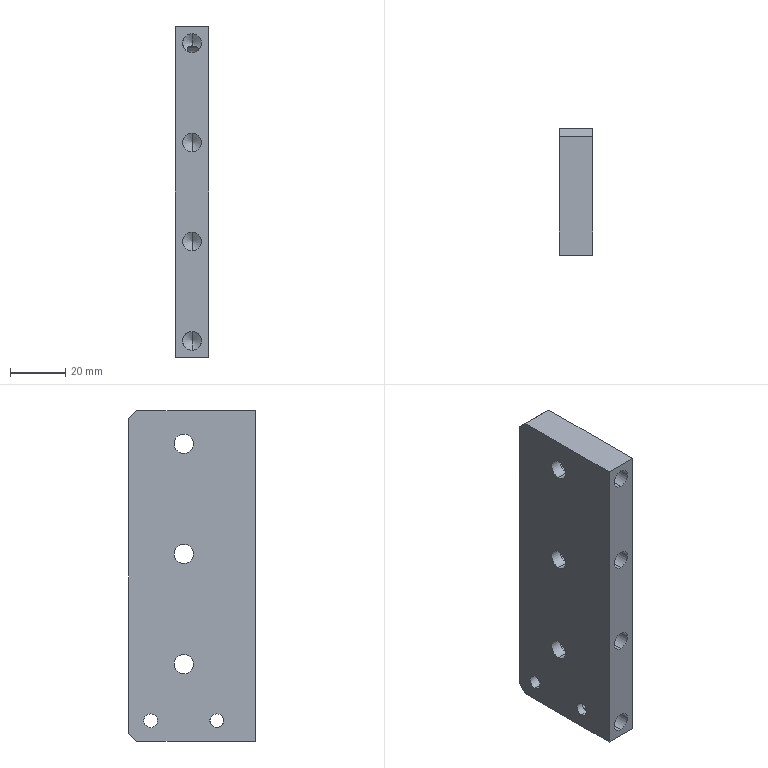Component | SolidWorks | ConveyorSideFixedLargePlateOne-2 | 1 solid | 43 faces | box 12 x 46 x 120 mm | volume 59730 mm3 | cylinder 24 | plane 11 | cone 8 | commonest cylinder face diameters 6.8 x8 11 x6 7 x6 5 x4 | material Plain Carbon Steel
build123d program:
from build123d import *

# Parameters (mm, degrees)
SKETCH1_W                                            = 120
SKETCH1_H                                            = 46
BOSS_EXTRUDE1_DEPTH                                  = 12
M8_TAPPED_HOLE1_D                                    = 6.8
M8_TAPPED_HOLE1_DEPTH                                = 22.25
M8_TAPPED_HOLE1_TIP                                  = 2.043
SKETCH4_R                                            = 3.5
CUT_EXTRUDE1_DEPTH                                   = 66.368
M6_TAPPED_HOLE1_D                                    = 5
HOLE_SIZE_ACCORDING_TO_TYPE_1_OF_HEXAGON_D           = 6.6
HOLE_SIZE_ACCORDING_TO_TYPE_1_OF_HEXAGON_CBORE_D     = 11
HOLE_SIZE_ACCORDING_TO_TYPE_1_OF_HEXAGON_CBORE_DEPTH = 7.8
CHAMFER1_SIZE                                        = 3


with BuildPart() as part:
    # Sketch1 → Boss-Extrude1 (new body)
    with BuildSketch(Plane(origin=(0, 0, 0), x_dir=(0, 0, -1), z_dir=(1, 0, 0))):
        Rectangle(SKETCH1_W, SKETCH1_H)
    extrude(amount=BOSS_EXTRUDE1_DEPTH)

    # M8 Tapped Hole1
    with Locations(Plane(origin=(0, -23, 0), x_dir=(-1, 0, 0), z_dir=(0, -1, 0))):
        with Locations((-6, 54), (-6, 18), (-6, -54), (-6, -18)):
            Hole(M8_TAPPED_HOLE1_D / 2, depth=M8_TAPPED_HOLE1_DEPTH)
            with Locations((0, 0, -(M8_TAPPED_HOLE1_DEPTH + M8_TAPPED_HOLE1_TIP / 2))):  # 118° drill point
                Cone(0, M8_TAPPED_HOLE1_D / 2, M8_TAPPED_HOLE1_TIP, mode=Mode.SUBTRACT)

    # Sketch4 → Cut-Extrude1 (cut, through all)
    with BuildSketch(Plane(origin=(12, 0, 0), x_dir=(0, 0, -1), z_dir=(1, 0, 0))):
        with Locations((-48, 3)):
            Circle(SKETCH4_R)
        with Locations((-8, 3)):
            Circle(SKETCH4_R)
        with Locations((32, 3)):
            Circle(SKETCH4_R)
    extrude(amount=-CUT_EXTRUDE1_DEPTH, mode=Mode.SUBTRACT)

    # M6 Tapped Hole1 (through all)
    with Locations(Plane.ZY):
        with Locations((-52.5, 15), (-52.5, -9)):
            Hole(M6_TAPPED_HOLE1_D / 2)

    # Hole Size according to type 1 of hexagon (through all)
    with Locations(Plane(origin=(12, -9.244, 5.634), x_dir=(0, 0, 1), z_dir=(1, 0, 0))):
        with Locations((-37.634, -12.244), (2.366, -12.244), (42.366, -12.244)):
            CounterBoreHole(HOLE_SIZE_ACCORDING_TO_TYPE_1_OF_HEXAGON_D / 2, HOLE_SIZE_ACCORDING_TO_TYPE_1_OF_HEXAGON_CBORE_D / 2, HOLE_SIZE_ACCORDING_TO_TYPE_1_OF_HEXAGON_CBORE_DEPTH)

    # Chamfer1
    chamfer1_edges = [part.edges().sort_by_distance(p)[0] for p in [
        (6, 23, 60),
        (6, 23, -60),
    ]]
    chamfer(chamfer1_edges, length=CHAMFER1_SIZE)


solid = part.part

# Placed as in the assembly
solid = solid.moved(Location((35.45, 2.646, 315), (0, 0, 0)))